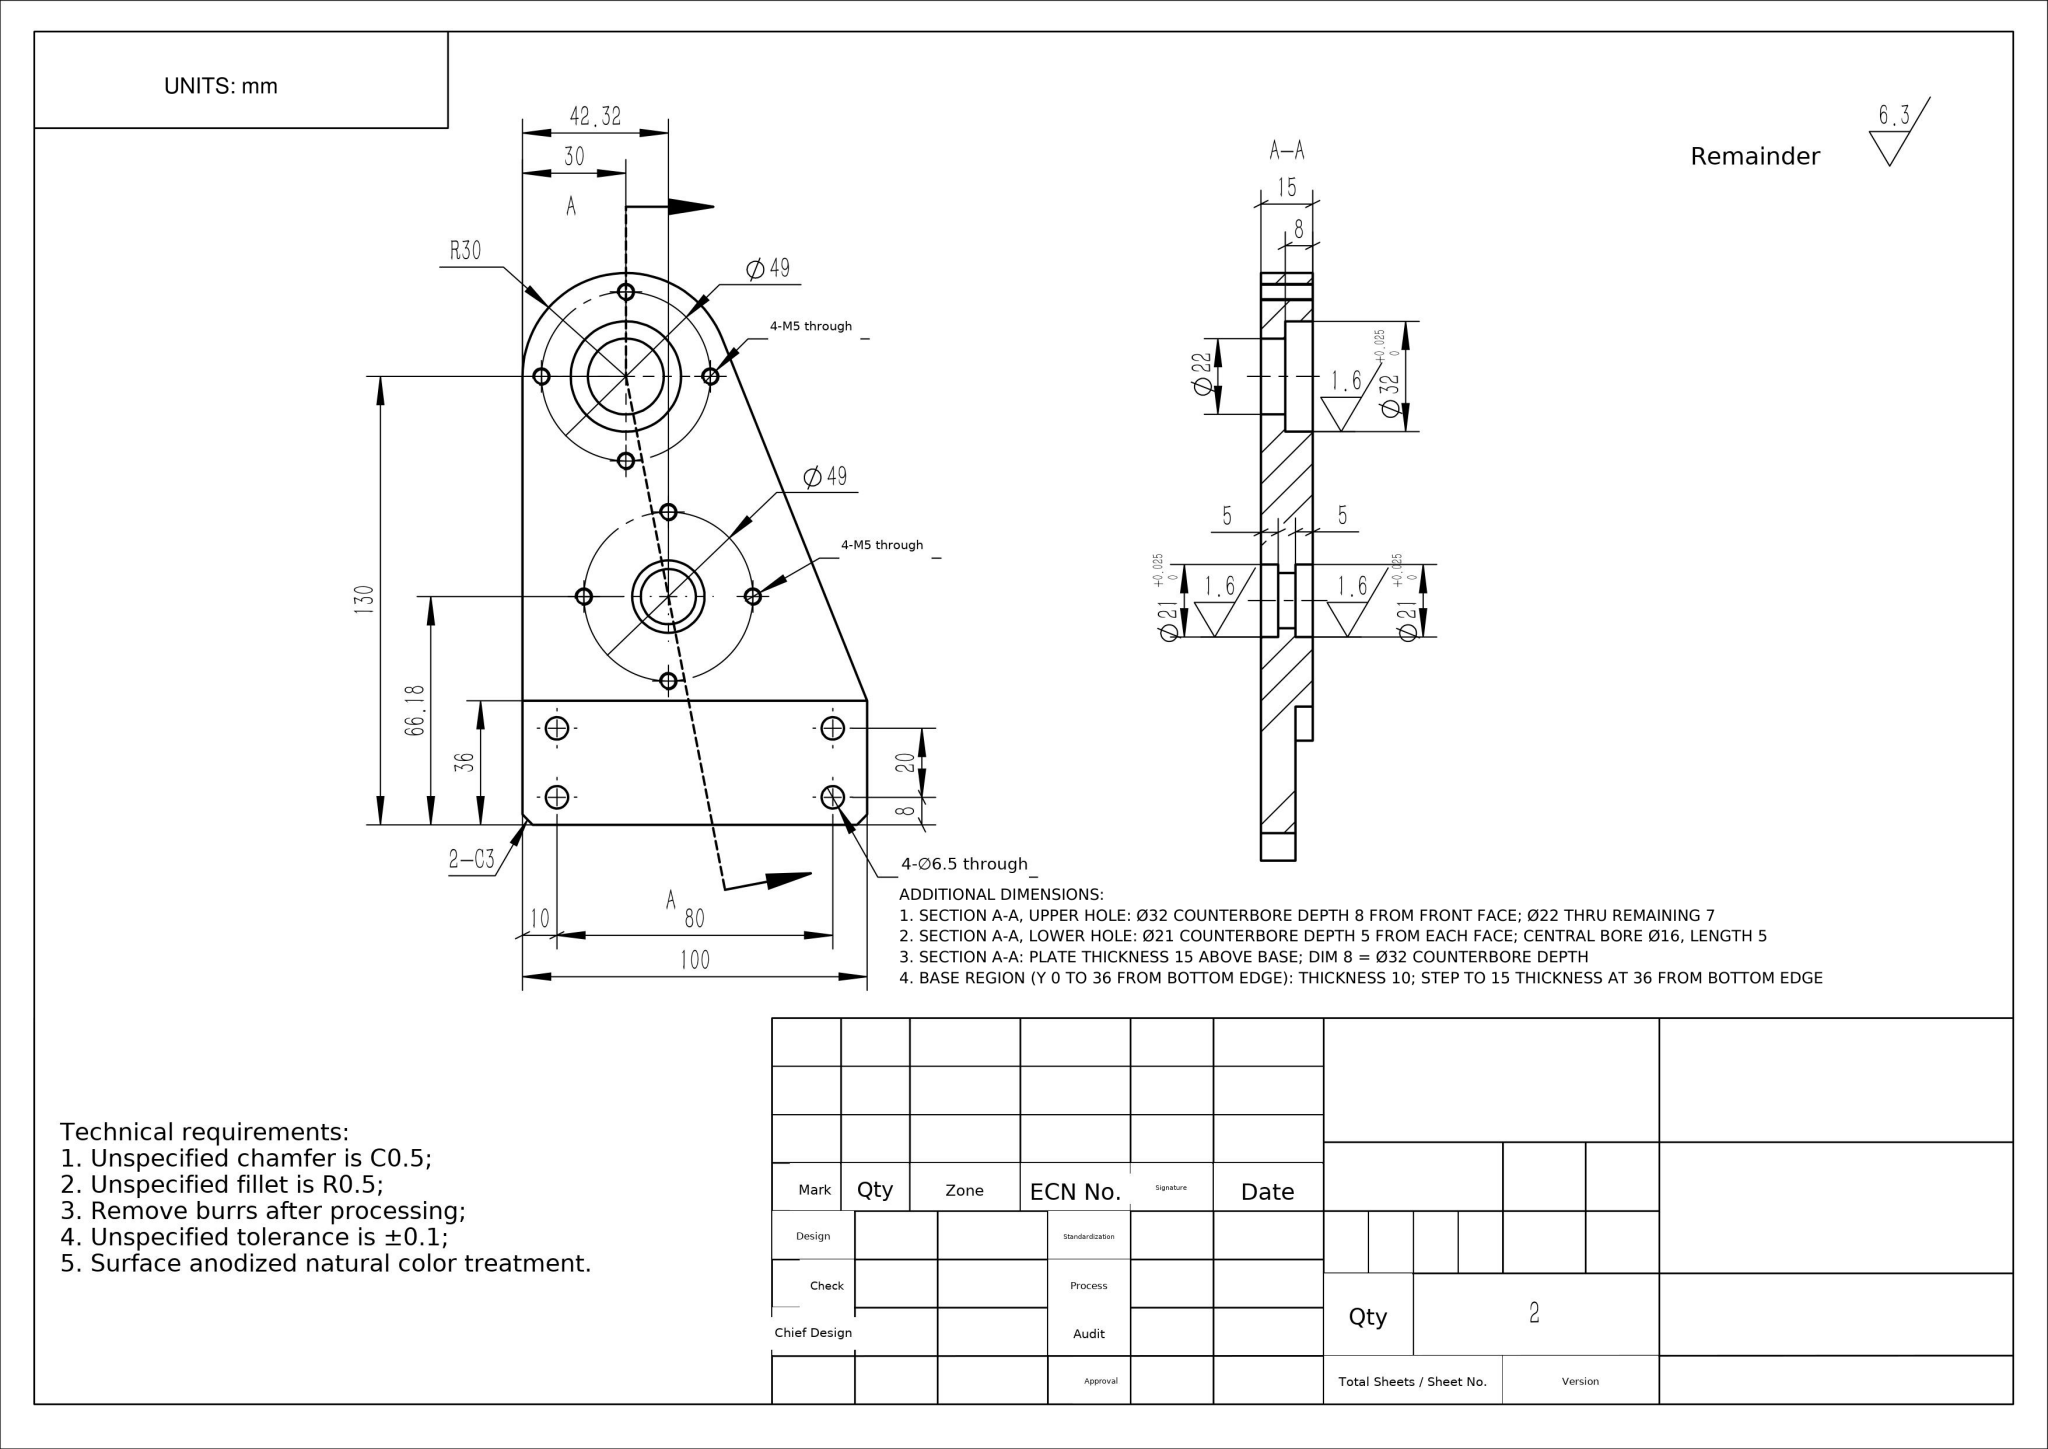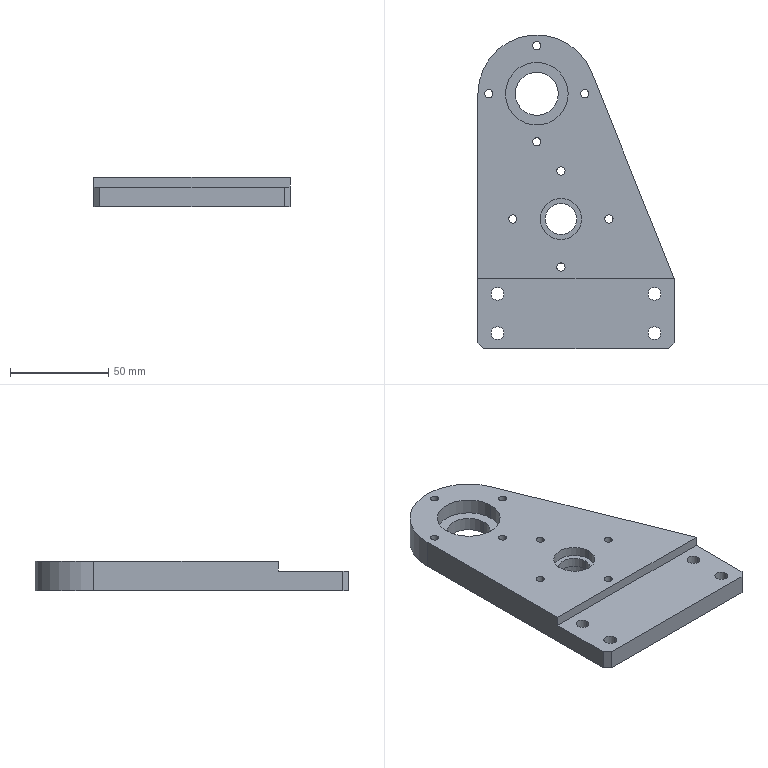Part | NX | mm | 1 solid | 48 faces | box 100 x 160 x 15 mm | volume 155130 mm3 | cylinder 35 | plane 13 | commonest cylinder face diameters 4.2 x16 6.5 x8 21 x4 32 x2 22 x2 16 x2 60 x1